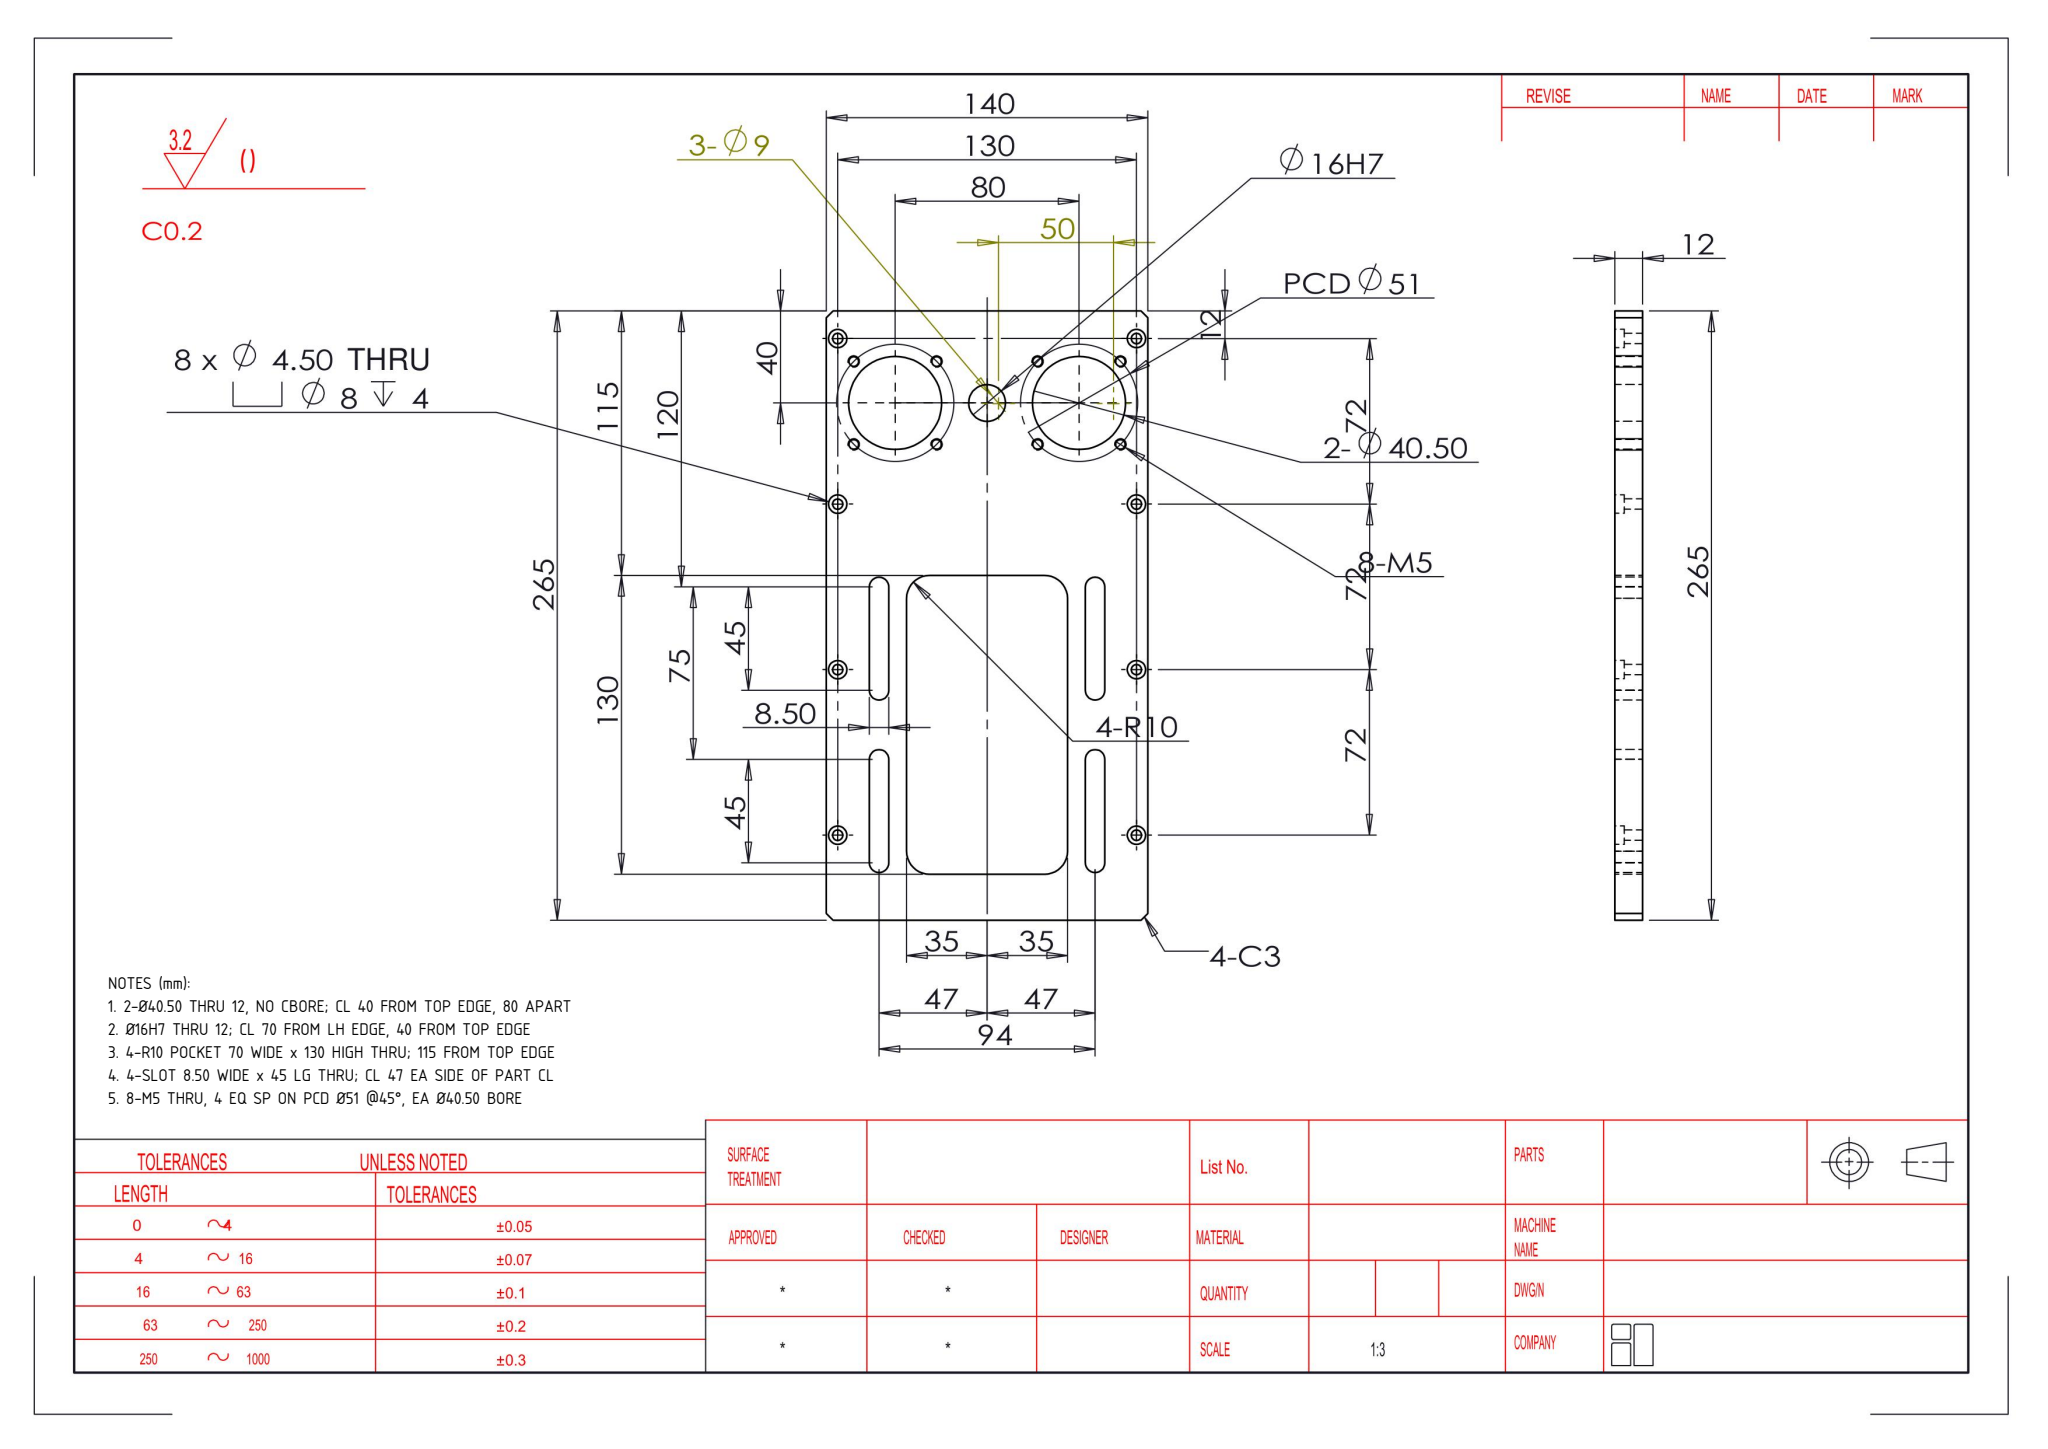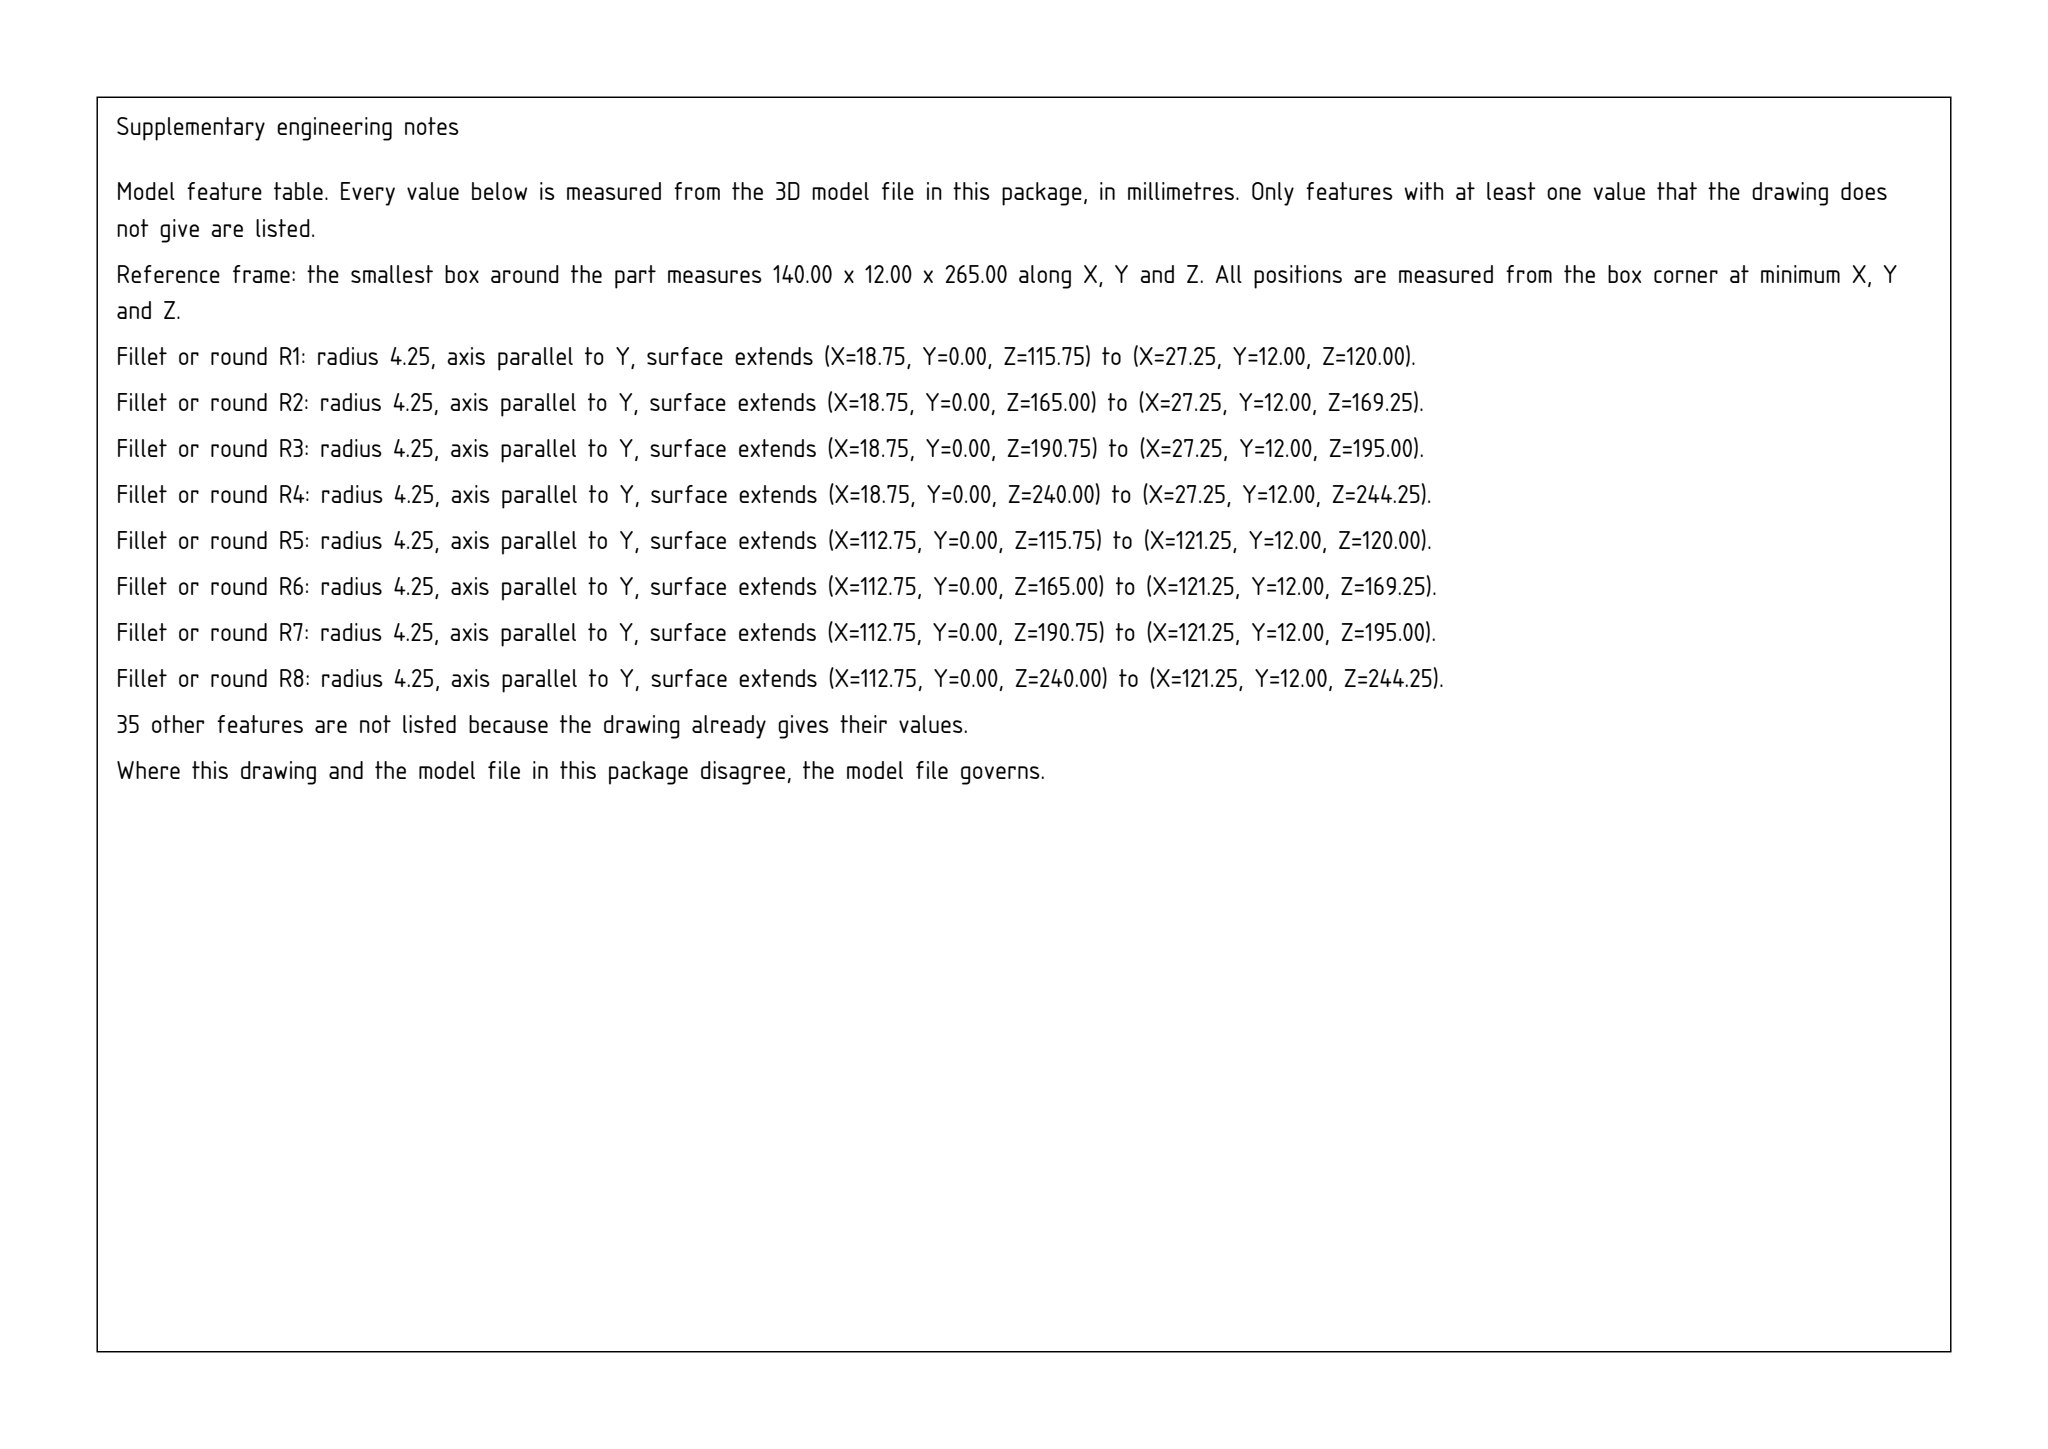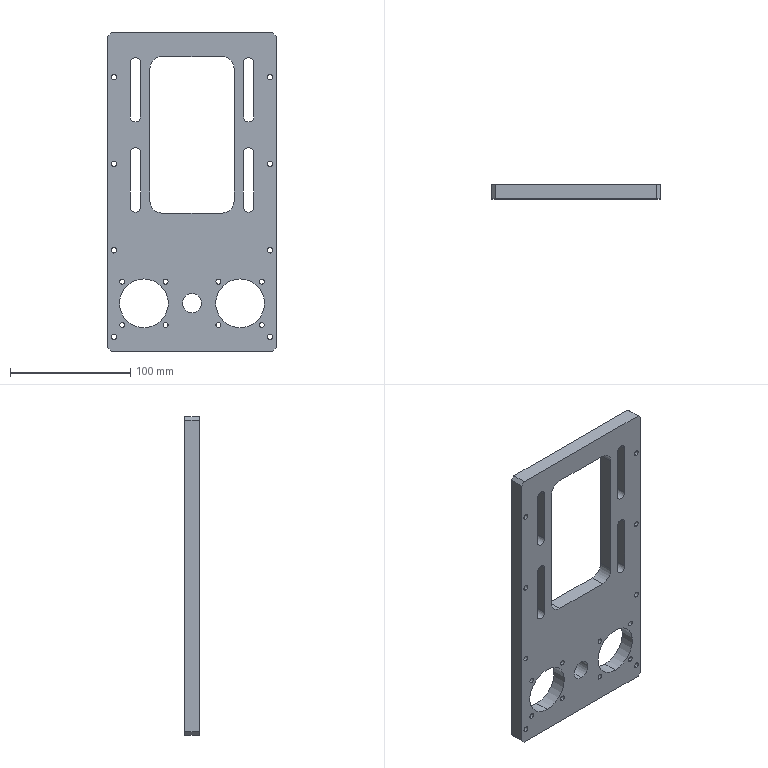Part | SolidWorks | mm | 1 solid | 100 faces | box 140 x 12 x 265 mm | volume 278443 mm3 | cylinder 70 | plane 30 | commonest cylinder face diameters 8 x16 4.5 x16 4.2 x16 8.5 x12 40.5 x4 20 x4 16 x2
Drawing notes:
2-Ø40.50 THRU 12, NO CBORE; CL 40 FROM TOP EDGE, 80 APART | from the solid: Ø40.5 cyls axis y at (30,40) & (110,40), length 12 = full plate thk; no intermediate y-plane
Ø16H7 THRU 12; CL 70 FROM LH EDGE, 40 FROM TOP EDGE | from the solid: Ø16 cyl axis y at (70,40), length 12 = full thk
4-R10 POCKET 70 WIDE x 130 HIGH THRU; 115 FROM TOP EDGE | from the solid: X-planes 35/105, Z-planes 115/245, R10 corner cyls Ø20 at (45,125),(95,125),(45,235),(95,235), 12 thk = thru
4-SLOT 8.50 WIDE x 45 LG THRU; CL 47 EA SIDE OF PART CL | from the solid: Ø8.5 cyls len 12 at x=23 & 117, z=120/165 and 195/240
8-M5 THRU, 4 EQ SP ON PCD Ø51 @45°, EA Ø40.50 BORE | from the solid: Ø4.2 tap-drill cyls len 12 (thru) at ±18.03 x/z from (30,40) and (110,40) = PCD 51 at 45°
build123d program:
from build123d import *

# Parameters (mm, degrees)
SKETCH1_W                                       = 140
SKETCH1_H                                       = 265
SKETCH1_R                                       = 20.25
SKETCH1_R_2                                     = 8
SKETCH1_W_2                                     = 70
SKETCH1_H_2                                     = 130
EXTRUDE1_DEPTH                                  = 12
FILLET1_R                                       = 10
EXTRUDE2_DEPTH                                  = 298.922
SKETCH5_R                                       = 1
EXTRUDE4_DEPTH                                  = 298.922
M5_TAPPED_HOLE1_D                               = 4.2
M4_HEX_SOCKET_HEAD_CAP_SCREW_CBORE1_D           = 4.5
M4_HEX_SOCKET_HEAD_CAP_SCREW_CBORE1_CBORE_D     = 8
M4_HEX_SOCKET_HEAD_CAP_SCREW_CBORE1_CBORE_DEPTH = 4
CHAMFER1_SIZE                                   = 3


with BuildPart() as part:
    # Sketch1 → Extrude1 (new body)
    with BuildSketch(Plane(origin=(0, 0, 0), x_dir=(1, 0, 0), z_dir=(0, 1, 0))):
        with Locations((35.05, 146.029)):
            Rectangle(SKETCH1_W, SKETCH1_H)
        with Locations(Location((-4.95, 238.529, 0), (0, 0, 270))):
            Circle(SKETCH1_R, mode=Mode.SUBTRACT)
        with Locations(Location((75.05, 238.529, 0), (0, 0, 270))):
            Circle(SKETCH1_R, mode=Mode.SUBTRACT)
        with Locations(Location((35.05, 238.529, 0), (0, 0, 270))):
            Circle(SKETCH1_R_2, mode=Mode.SUBTRACT)
        with Locations((35.05, 98.529)):
            Rectangle(SKETCH1_W_2, SKETCH1_H_2, mode=Mode.SUBTRACT)
    extrude(amount=EXTRUDE1_DEPTH)

    # Fillet1
    fillet1_edges = [part.edges().sort_by_distance(p)[0] for p in [
        (0.05031, 6, -163.529),
        (0.05031, 6, -33.529),
        (70.05, 6, -33.529),
        (70.05, 6, -163.529),
    ]]
    fillet(fillet1_edges, radius=FILLET1_R)

    # Sketch2 → Extrude2 (cut, through all)
    with BuildSketch(Plane(origin=(0, 12, 0), x_dir=(-1, 0, 0), z_dir=(0, 1, 0))):
        with BuildLine():
            Line((-86.3, -83.529), (-86.3, -38.529))
            ThreePointArc((-86.3, -38.529), (-82.05, -34.279), (-77.8, -38.529))
            Line((-77.8, -38.529), (-77.8, -83.529))
            ThreePointArc((-77.8, -83.529), (-82.05, -87.779), (-86.3, -83.529))
        make_face()
        with BuildLine():
            Line((16.2, -158.529), (16.2, -113.529))
            ThreePointArc((16.2, -113.529), (11.95, -109.279), (7.7, -113.529))
            Line((7.7, -113.529), (7.7, -158.529))
            ThreePointArc((7.7, -158.529), (11.95, -162.779), (16.2, -158.529))
        make_face()
        with BuildLine():
            Line((7.7, -83.529), (7.7, -38.529))
            ThreePointArc((7.7, -38.529), (11.95, -34.279), (16.2, -38.529))
            Line((16.2, -38.529), (16.2, -83.529))
            ThreePointArc((16.2, -83.529), (11.95, -87.779), (7.7, -83.529))
        make_face()
        with BuildLine():
            Line((-77.8, -158.529), (-77.8, -113.529))
            ThreePointArc((-77.8, -113.529), (-82.05, -109.279), (-86.3, -113.529))
            Line((-86.3, -113.529), (-86.3, -158.529))
            ThreePointArc((-86.3, -158.529), (-82.05, -162.779), (-77.8, -158.529))
        make_face()
    extrude(amount=-EXTRUDE2_DEPTH, mode=Mode.SUBTRACT)

    # Sketch5 → Extrude4 (cut, through all)
    with BuildSketch(Plane(origin=(0, 12, 0), x_dir=(-1, 0, 0), z_dir=(0, 1, 0))):
        with Locations(Location((-13.082, -220.497, 0), (0, 0, 90))):
            Circle(SKETCH5_R)
        with Locations(Location((-57.019, -220.497, 0), (0, 0, 90))):
            Circle(SKETCH5_R)
        with Locations(Location((22.981, -220.497, 0), (0, 0, 90))):
            Circle(SKETCH5_R)
        with Locations(Location((22.981, -256.56, 0), (0, 0, 90))):
            Circle(SKETCH5_R)
        with Locations(Location((-13.082, -256.56, 0), (0, 0, 90))):
            Circle(SKETCH5_R)
        with Locations(Location((-57.019, -256.56, 0), (0, 0, 90))):
            Circle(SKETCH5_R)
        with Locations(Location((-93.082, -256.56, 0), (0, 0, 90))):
            Circle(SKETCH5_R)
        with Locations(Location((-93.082, -220.497, 0), (0, 0, 90))):
            Circle(SKETCH5_R)
    extrude(amount=-EXTRUDE4_DEPTH, mode=Mode.SUBTRACT)

    # M5 Tapped Hole1 (through all)
    with Locations(Plane(origin=(-22.981, 12, -256.56), x_dir=(0, 0, 1), z_dir=(0, 1, 0))):
        with Locations((0, 0), (0, 36.062), (36.062, 0), (36.062, 36.062), (0, 116.062), (0, 80), (36.062, 80), (36.062, 116.062)):
            Hole(M5_TAPPED_HOLE1_D / 2)

    # M4 Hex Socket Head Cap Screw CBORE1 (through all)
    with Locations(Plane(origin=(100.05, 12, -266.529), x_dir=(0, 0, 1), z_dir=(0, 1, 0))):
        with Locations((0, 0), (72, 0), (144, 0), (216, 0), (216, -130), (144, -130), (72, -130), (0, -130)):
            CounterBoreHole(M4_HEX_SOCKET_HEAD_CAP_SCREW_CBORE1_D / 2, M4_HEX_SOCKET_HEAD_CAP_SCREW_CBORE1_CBORE_D / 2, M4_HEX_SOCKET_HEAD_CAP_SCREW_CBORE1_CBORE_DEPTH)

    # Chamfer1
    chamfer1_edges = [part.edges().sort_by_distance(p)[0] for p in [
        (-34.95, 6, -278.529),
        (105.05, 6, -278.529),
        (105.05, 6, -13.529),
        (-34.95, 6, -13.529),
    ]]
    chamfer(chamfer1_edges, length=CHAMFER1_SIZE)


solid = part.part